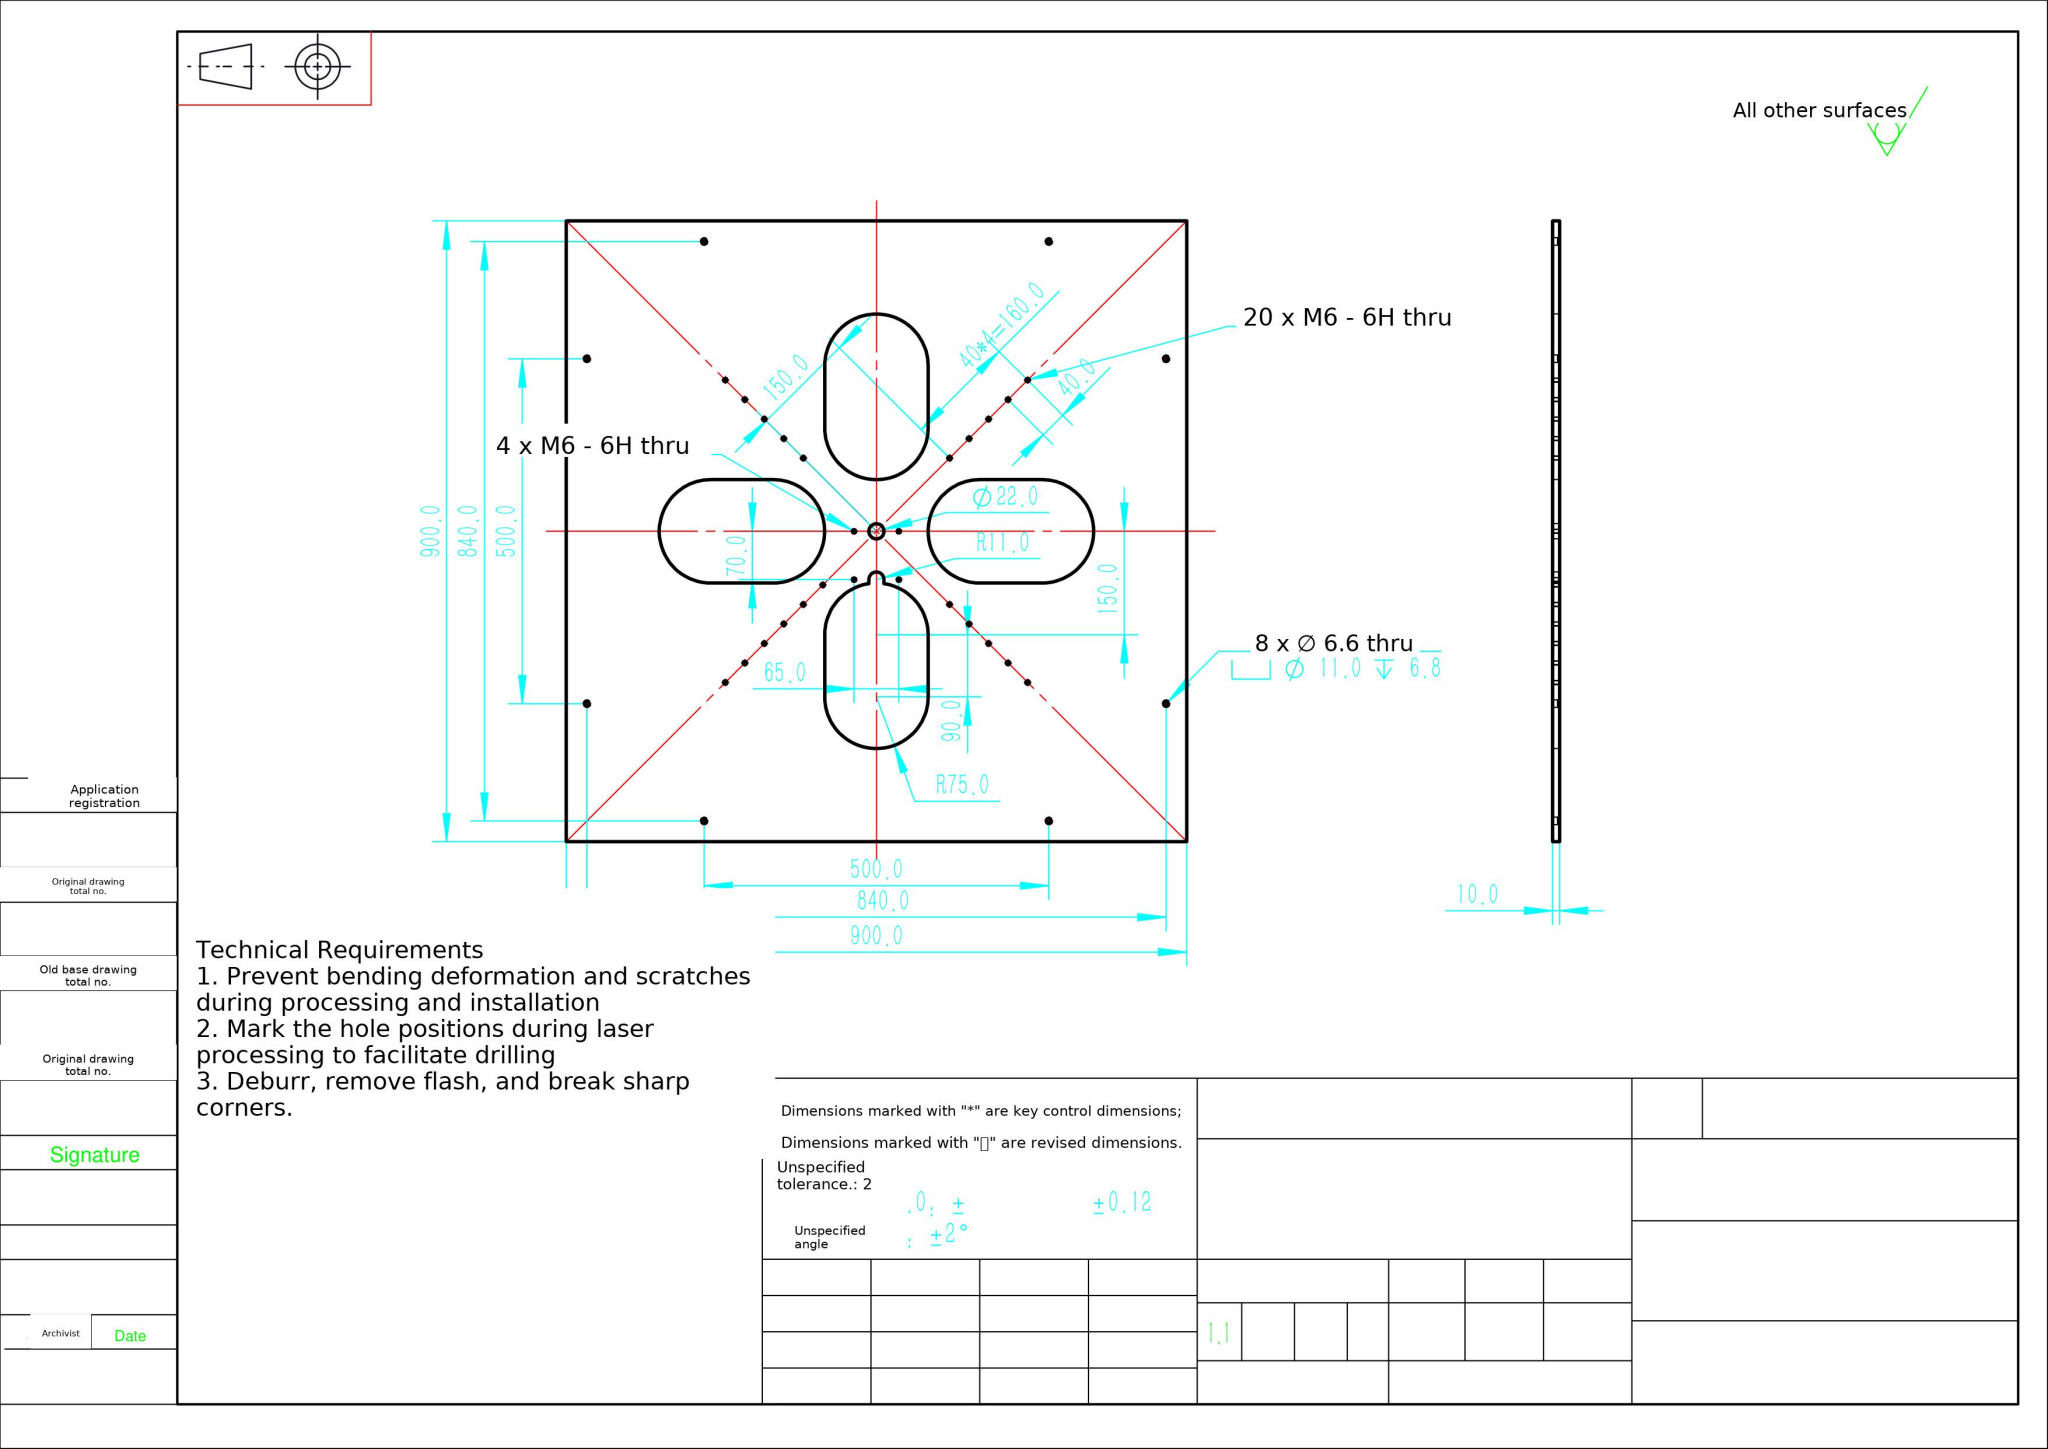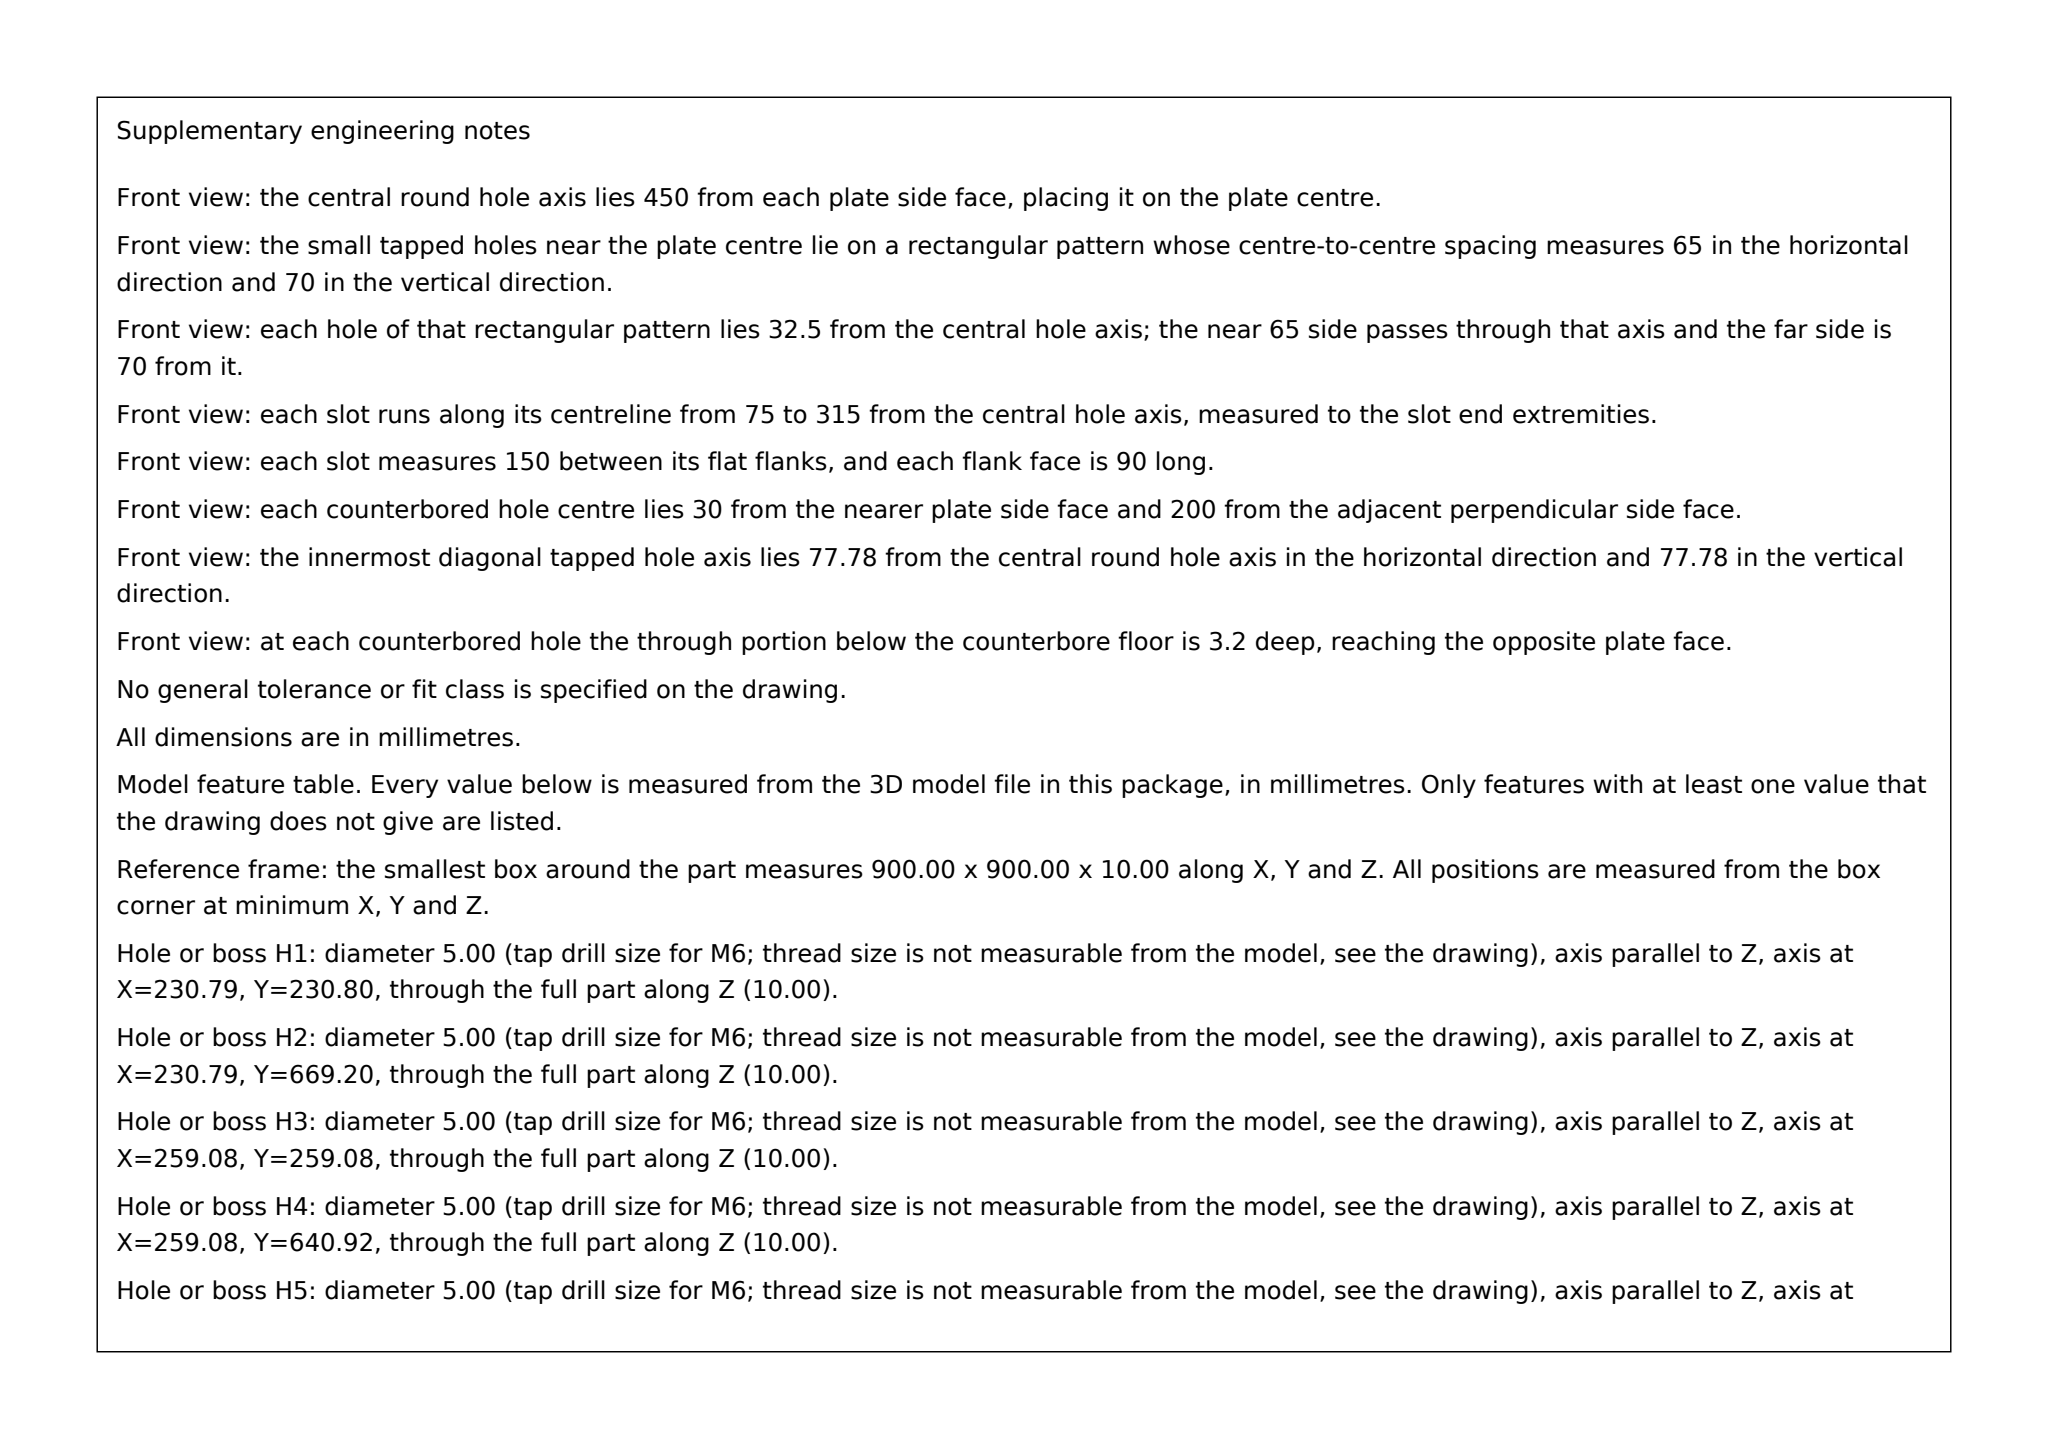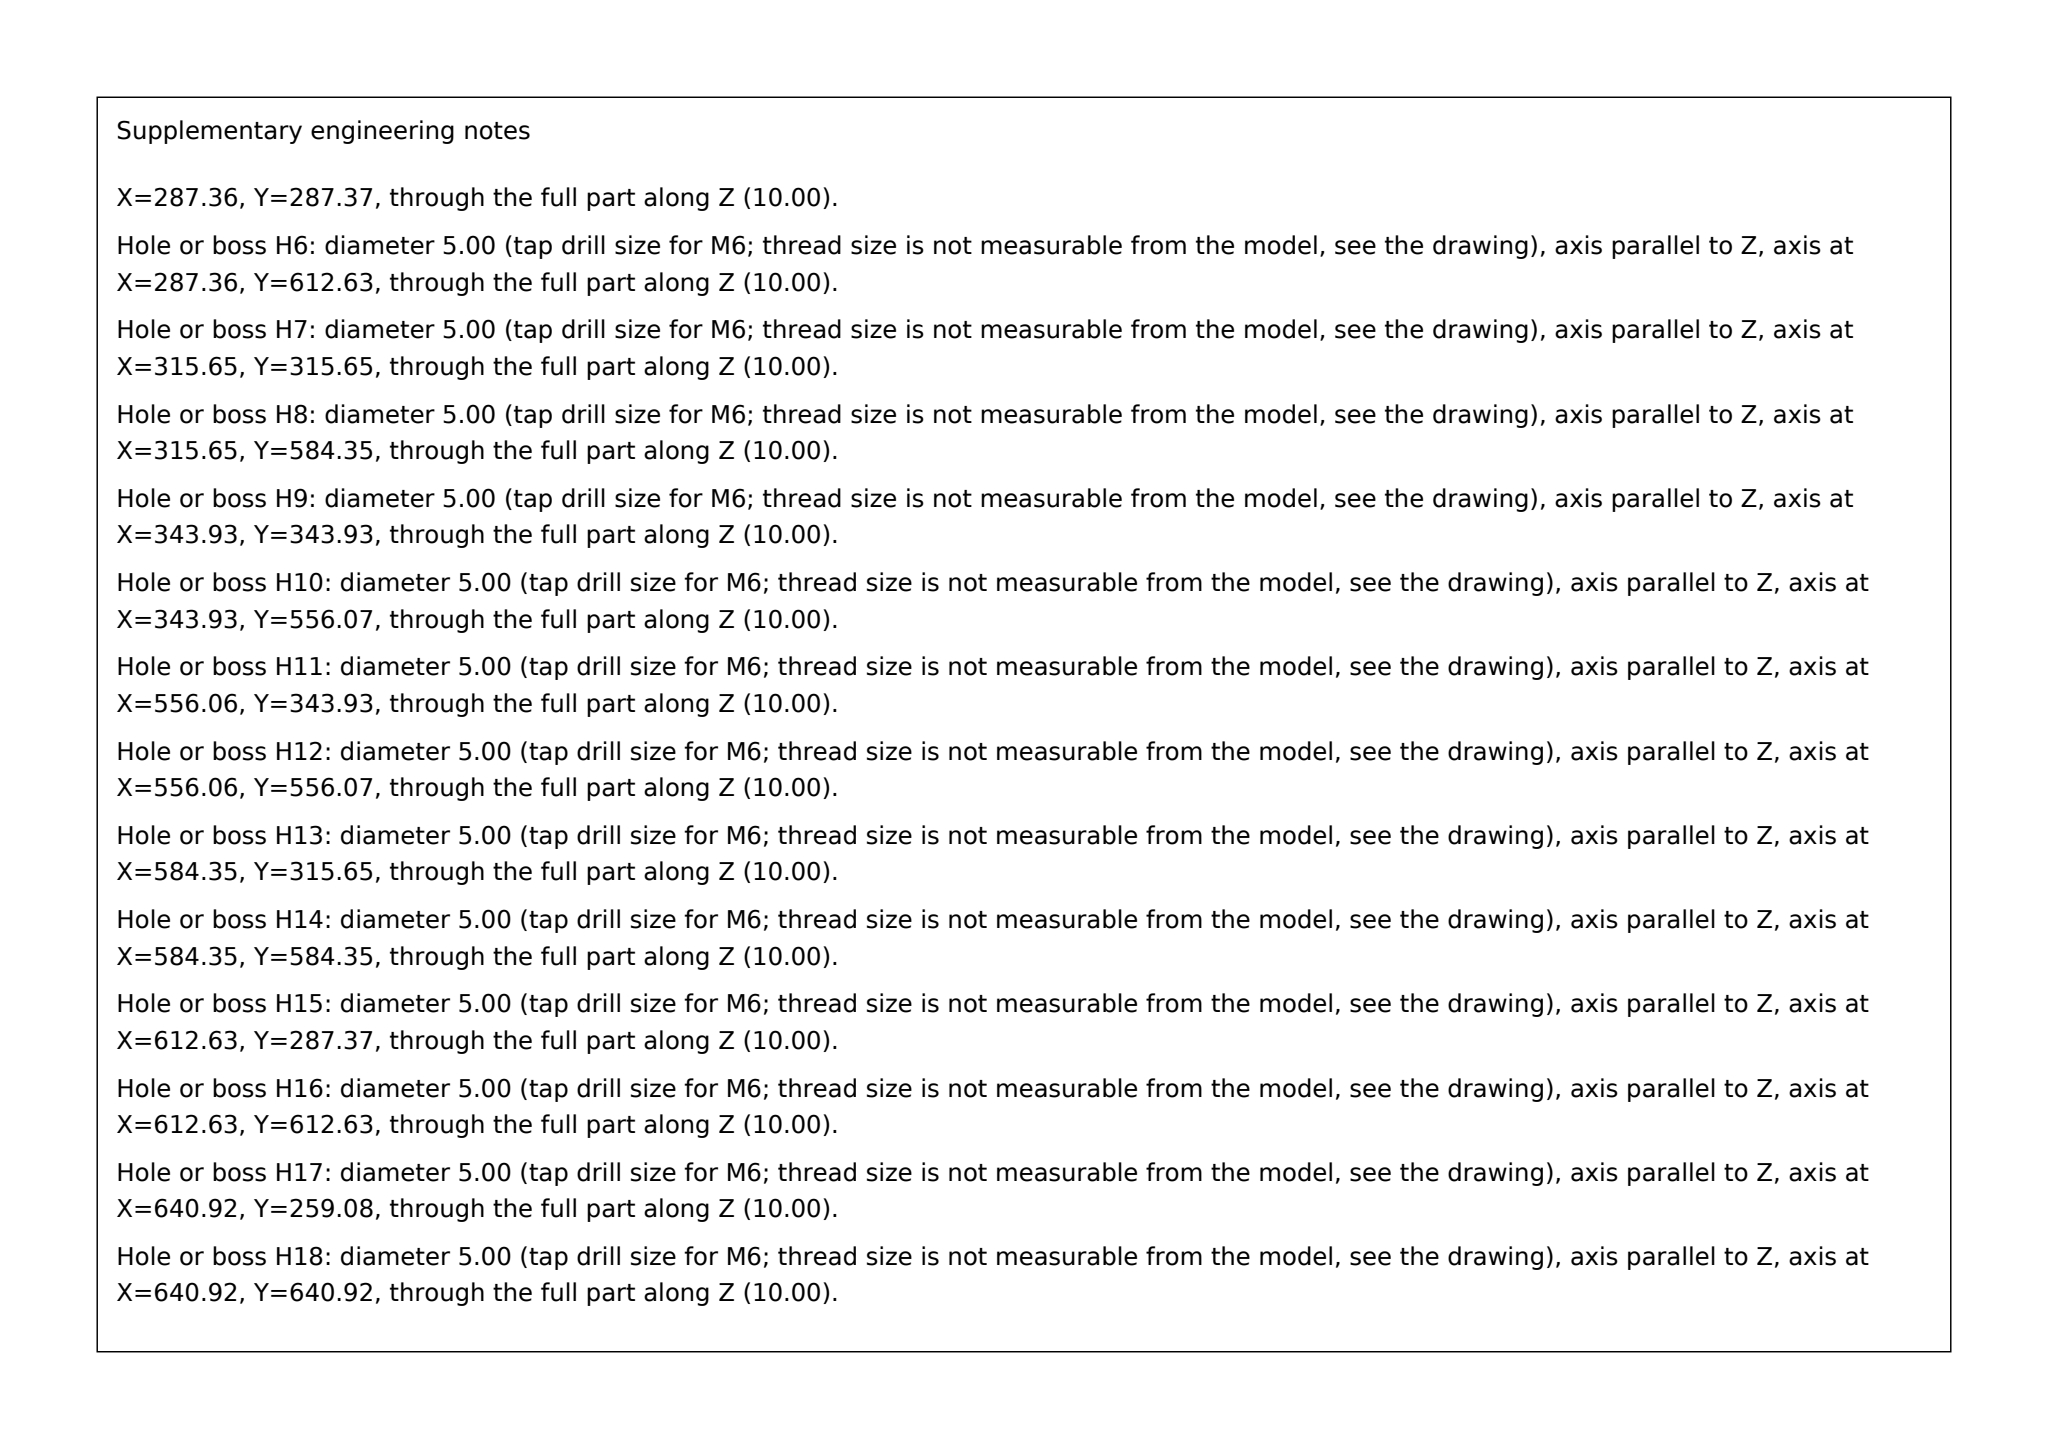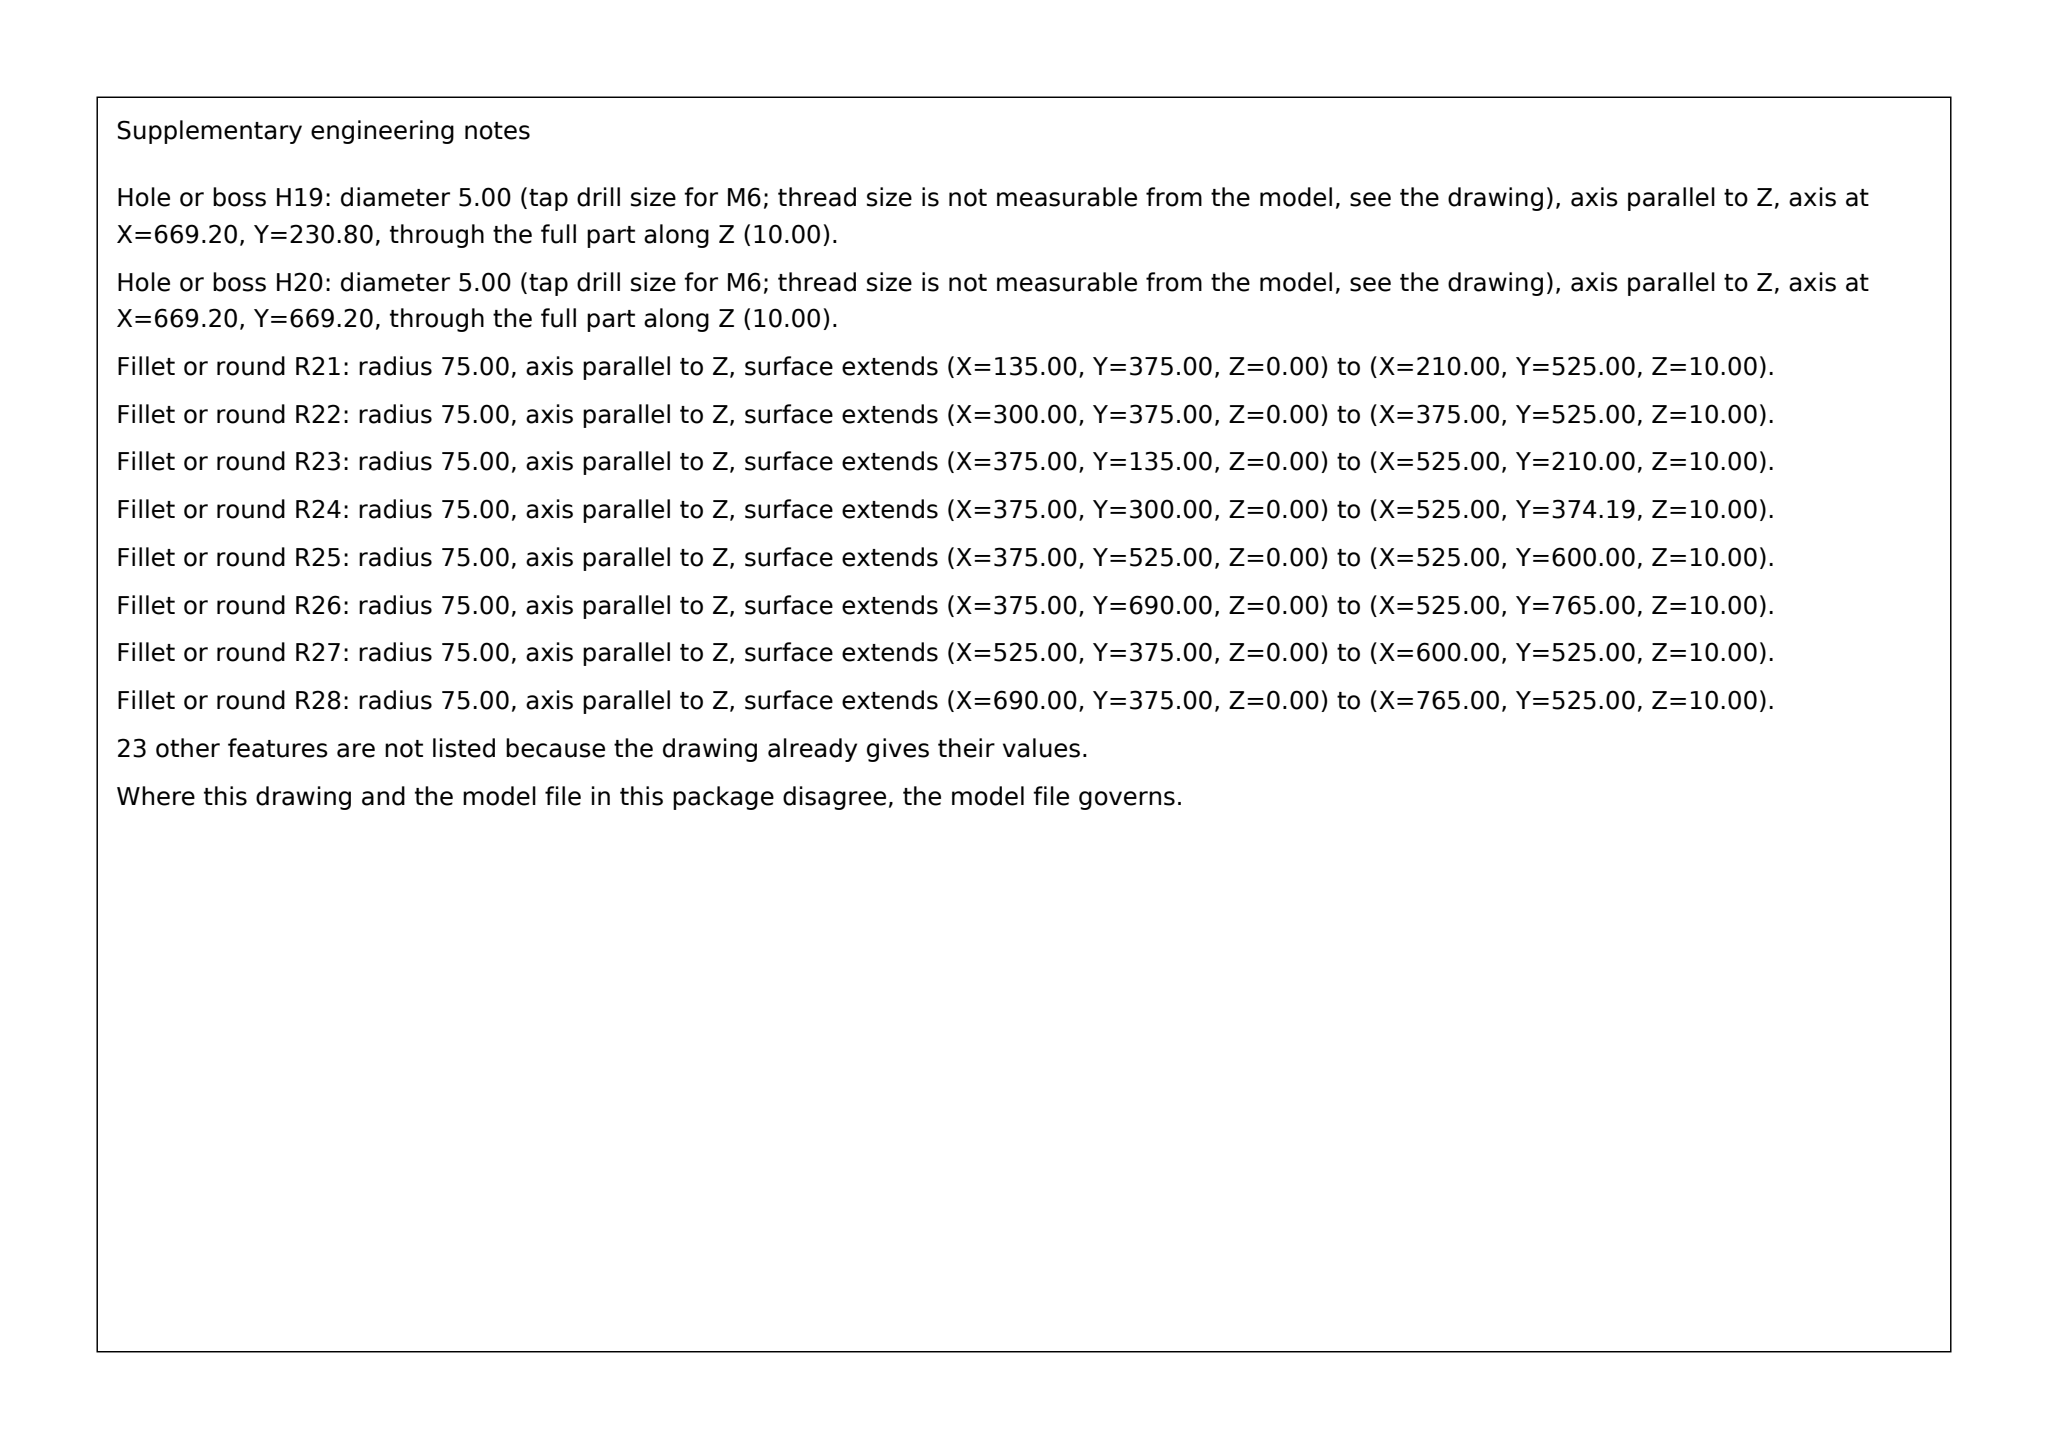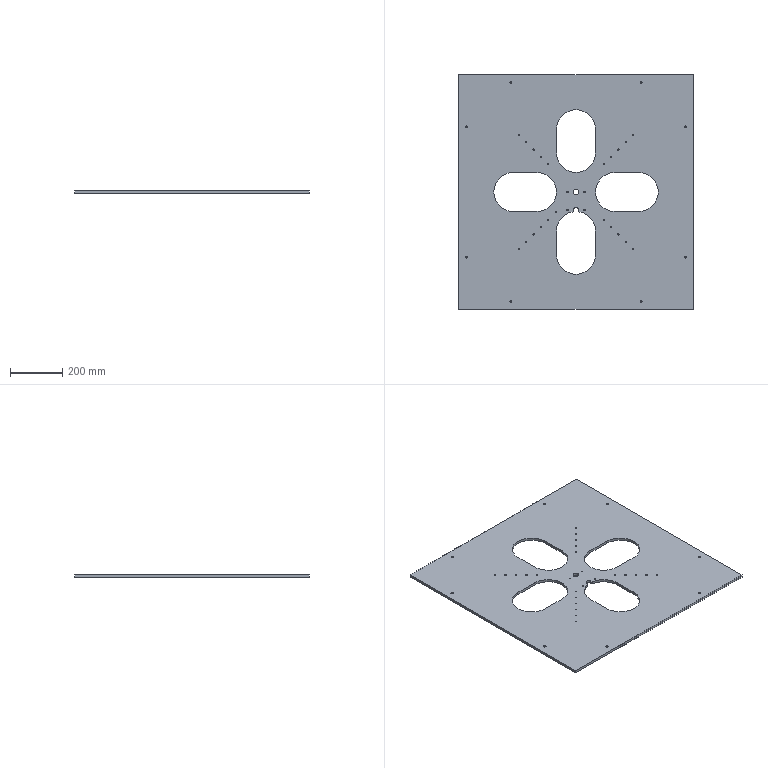Part | SolidWorks | mm | 1 solid | 121 faces | box 900 x 900 x 10 mm | volume 6835326 mm3 | cylinder 97 | plane 24 | commonest cylinder face diameters 5 x50 11 x16 6.6 x16 150 x11 22 x4
Drawing notes:
4X OBROUND SLOT: 150 WIDE X 240 OVERALL LENGTH, R75 ENDS, 90 CENTER-TO-CENTER OF END RADII, THRU 10 PLATE | from the solid: Ø150 z-cylinders paired at (450,600)&(450,690); (450,210)&(450,300); (210,450)&(300,450); (600,450)&(690,450), length 10 = plate thickness
SLOT LOCATIONS FROM PLATE CENTER (450,450 FROM MIN CORNER OF 900X900 PLATE): SLOT CENTERS AT 195 FROM CENTER ON X AND Y AXES, i.e. (255,450), (645,450), (450,255), (450,645) | from the solid: Ø150 end-radii centers midpoints: (255,450),(645,450),(450,255),(450,645) vs bbox 900x900 center (450,450)
4X M6-6H LOCATED AT X=417.5 AND X=482.5 (65 APART, SYMMETRIC ±32.5 ABOUT PLATE CENTERLINE), ON Y=450 (PLATE CENTERLINE) AND Y=380 (70 BELOW CENTERLINE) | from the solid: Ø5.0 z-cylinders at (417.5,450),(482.5,450),(417.55,380),(482.55,380)
20X M6-6H ON FOUR 45° DIAGONALS FROM PLATE CENTER: 5 HOLES PER DIAGONAL, 40 PITCH ALONG DIAGONAL, FIRST HOLE 150 AND LAST HOLE 310 RADIALLY FROM PLATE CENTER | from the solid: Ø5.0 z-cylinders at (343.93,343.93),(315.65,315.65),(287.37,287.37),(259.08,259.08),(230.8,230.8) and the three mirrored diagonal sets; radial distances 150,190,230,270,310 from (450,450)
ALL M6-6H HOLES THRU (10 DEEP, FULL PLATE THICKNESS) | from the solid: Ø5.0 cylinders length 10.0 = bbox Z 10.0
ALL DIMENSIONS IN MILLIMETERS | from the solid: STEP model units mm; bbox_xyz 900.0 x 900.0 x 10.0
1X ADDITIONAL M6-6H THRU (10 DEEP, FULL THICKNESS) AT X=372.22, Y=372.22 FROM PLATE MIN CORNER = R110 FROM PLATE CENTER (450,450) ON LOWER-LEFT 45° DIAGONAL | from the solid: cylinders: [5.0, z, (372.22, 372.22), length 10.0] - tapped M6 minor-dia hole thru 10 plate
TOTAL TAPPED HOLE COUNT IS 21X M6-6H ON THE 45° DIAGONALS: 5 HOLES (R150, 190, 230, 270, 310) ON EACH OF FOUR DIAGONALS PLUS 1 HOLE AT R110 ON THE LOWER-LEFT DIAGONAL | from the solid: cylinders dia 5.0 axis z: 20 holes at R150-R310 on four diagonals (e.g. 230.8/230.8 ... 669.2/669.2) plus (372.22,372.22) at R110
2X Ø22.0 (R11.0) THRU, 10 DEEP (FULL PLATE THICKNESS): ONE AT PLATE CENTER X=450, Y=450 AND ONE AT X=450, Y=380 (70 BELOW PLATE CENTERLINE), DIMENSIONED FROM PLATE MIN CORNER OF 900X900 PLATE | from the solid: cylinders [22.0,"z",[450.0,450.0],10.0] and [22.0,"z",[450.0,380.0],10.0]; bbox_xyz 900x900x10
build123d program:
from build123d import *

# Parameters (mm, degrees)
SKETCH1_W                                         = 2700
SKETCH1_H                                         = 900
SKETCH1_R                                         = 6.25
BOSS_EXTRUDE1_DEPTH                               = 10
SKETCH3_R                                         = 11
CUT_EXTRUDE2_DEPTH                                = 74
CUT_EXTRUDE3_DEPTH                                = 267
SKETCH5_W                                         = 1800
SKETCH5_H                                         = 900
CUT_EXTRUDE4_DEPTH                                = 10
HOLE_SIZE_ACCORDING_TO_TYPE_OF_HEXAGO_D           = 6.6
HOLE_SIZE_ACCORDING_TO_TYPE_OF_HEXAGO_CBORE_D     = 11
HOLE_SIZE_ACCORDING_TO_TYPE_OF_HEXAGO_CBORE_DEPTH = 6.8
M6_TAPPED_HOLE1_D                                 = 5
CUT_EXTRUDE5_REACH                                = 2156.168
M6_TAPPED_HOLE2_D                                 = 5


with BuildPart() as part:
    # Sketch1 → Boss-Extrude1 (new body)
    with BuildSketch(Plane.XY):
        with Locations((-613.954, 435)):
            Rectangle(SKETCH1_W, SKETCH1_H)
        with Locations((646.046, 75)):
            Circle(SKETCH1_R, mode=Mode.SUBTRACT)
        with Locations((-73.954, 795)):
            Circle(SKETCH1_R, mode=Mode.SUBTRACT)
        with Locations((646.046, 795)):
            Circle(SKETCH1_R, mode=Mode.SUBTRACT)
        with Locations((-73.954, 75)):
            Circle(SKETCH1_R, mode=Mode.SUBTRACT)
    extrude(amount=BOSS_EXTRUDE1_DEPTH)

    # Sketch3 → Cut-Extrude2 (cut)
    with BuildSketch(Plane.XY.offset(10)):
        with Locations((-1513.954, 435)):
            Circle(SKETCH3_R)
    extrude(amount=-CUT_EXTRUDE2_DEPTH, mode=Mode.SUBTRACT)

    # Sketch4 → Cut-Extrude3 (cut)
    with BuildSketch(Plane(origin=(0, 0, 0), x_dir=(-1, 0, 0), z_dir=(0, 0, -1))):
        with BuildLine():
            Line((1588.954, 195), (1588.954, 285))
            ThreePointArc((1588.954, 285), (1513.954, 360), (1438.954, 285))
            Line((1438.954, 285), (1438.954, 195))
            ThreePointArc((1438.954, 195), (1513.954, 120), (1588.954, 195))
        make_face()
        with BuildLine():
            Line((1273.954, 360), (1363.954, 360))
            ThreePointArc((1363.954, 360), (1438.954, 435), (1363.954, 510))
            Line((1363.954, 510), (1273.954, 510))
            ThreePointArc((1273.954, 510), (1198.954, 435), (1273.954, 360))
        make_face()
        with BuildLine():
            Line((1438.954, 675), (1438.954, 585))
            ThreePointArc((1438.954, 585), (1513.954, 510), (1588.954, 585))
            Line((1588.954, 585), (1588.954, 675))
            ThreePointArc((1588.954, 675), (1513.954, 750), (1438.954, 675))
        make_face()
        with BuildLine():
            Line((1753.954, 510), (1663.954, 510))
            ThreePointArc((1663.954, 510), (1588.954, 435), (1663.954, 360))
            Line((1663.954, 360), (1753.954, 360))
            ThreePointArc((1753.954, 360), (1828.954, 435), (1753.954, 510))
        make_face()
    extrude(amount=-CUT_EXTRUDE3_DEPTH, mode=Mode.SUBTRACT)

    # Sketch5 → Cut-Extrude4 (cut)
    with BuildSketch(Plane(origin=(0, 0, 0), x_dir=(-1, 0, 0), z_dir=(0, 0, -1))):
        with Locations((163.954, 435)):
            Rectangle(SKETCH5_W, SKETCH5_H)
    extrude(amount=-CUT_EXTRUDE4_DEPTH, mode=Mode.SUBTRACT)

    # Hole Size _ according to_ type of Hexago (through all)
    with Locations(Plane(origin=(0, 0, 0), x_dir=(-1, 0, 0), z_dir=(0, 0, -1))):
        with Locations((1263.954, 15), (1763.954, 15), (1933.954, 185), (1933.954, 685), (1763.954, 855), (1263.954, 855), (1093.954, 685), (1093.954, 185)):
            CounterBoreHole(HOLE_SIZE_ACCORDING_TO_TYPE_OF_HEXAGO_D / 2, HOLE_SIZE_ACCORDING_TO_TYPE_OF_HEXAGO_CBORE_D / 2, HOLE_SIZE_ACCORDING_TO_TYPE_OF_HEXAGO_CBORE_DEPTH)

    # M6 Tapped Hole1 (through all)
    with Locations(Plane(origin=(0, 0, 0), x_dir=(-1, 0, 0), z_dir=(0, 0, -1))):
        with Locations((1591.735, 357.218), (1620.02, 328.934), (1648.304, 300.65), (1676.588, 272.365), (1704.872, 244.081), (1733.157, 215.797), (1407.888, 328.934), (1379.603, 300.65), (1351.319, 272.365), (1323.035, 244.081), (1294.75, 215.797), (1407.888, 541.066), (1379.603, 569.35), (1351.319, 597.635), (1323.035, 625.919), (1294.75, 654.203), (1620.02, 541.066), (1648.304, 569.35), (1676.588, 597.635), (1704.872, 625.919), (1733.157, 654.203)):
            Hole(M6_TAPPED_HOLE1_D / 2)

    # Sketch10 → Cut-Extrude5 (cut, up to next)
    with BuildSketch(Plane(origin=(0, 0, 0), x_dir=(-1, 0, 0), z_dir=(0, 0, -1)), mode=Mode.PRIVATE) as cut_extrude5_sk1:
        with BuildLine():
            Line((1524.954, 365), (1524.954, 320.745))
            ThreePointArc((1524.954, 320.745), (1513.954, 309.745), (1502.954, 320.745))
            Line((1502.954, 320.745), (1502.954, 365))
            ThreePointArc((1502.954, 365), (1513.954, 376), (1524.954, 365))
        make_face()
    cut_extrude5_tool1 = extrude(cut_extrude5_sk1.sketch, amount=-CUT_EXTRUDE5_REACH, mode=Mode.PRIVATE) & part.part
    add(cut_extrude5_tool1.solids().sort_by_distance((-1513.954, 342.873, 0))[0], mode=Mode.SUBTRACT)

    # M6 Tapped Hole2 (through all)
    with Locations(Plane.XY.offset(10)):
        with Locations((-1546.408, 365), (-1481.408, 365), (-1481.454, 435), (-1546.454, 435)):
            Hole(M6_TAPPED_HOLE2_D / 2)


solid = part.part